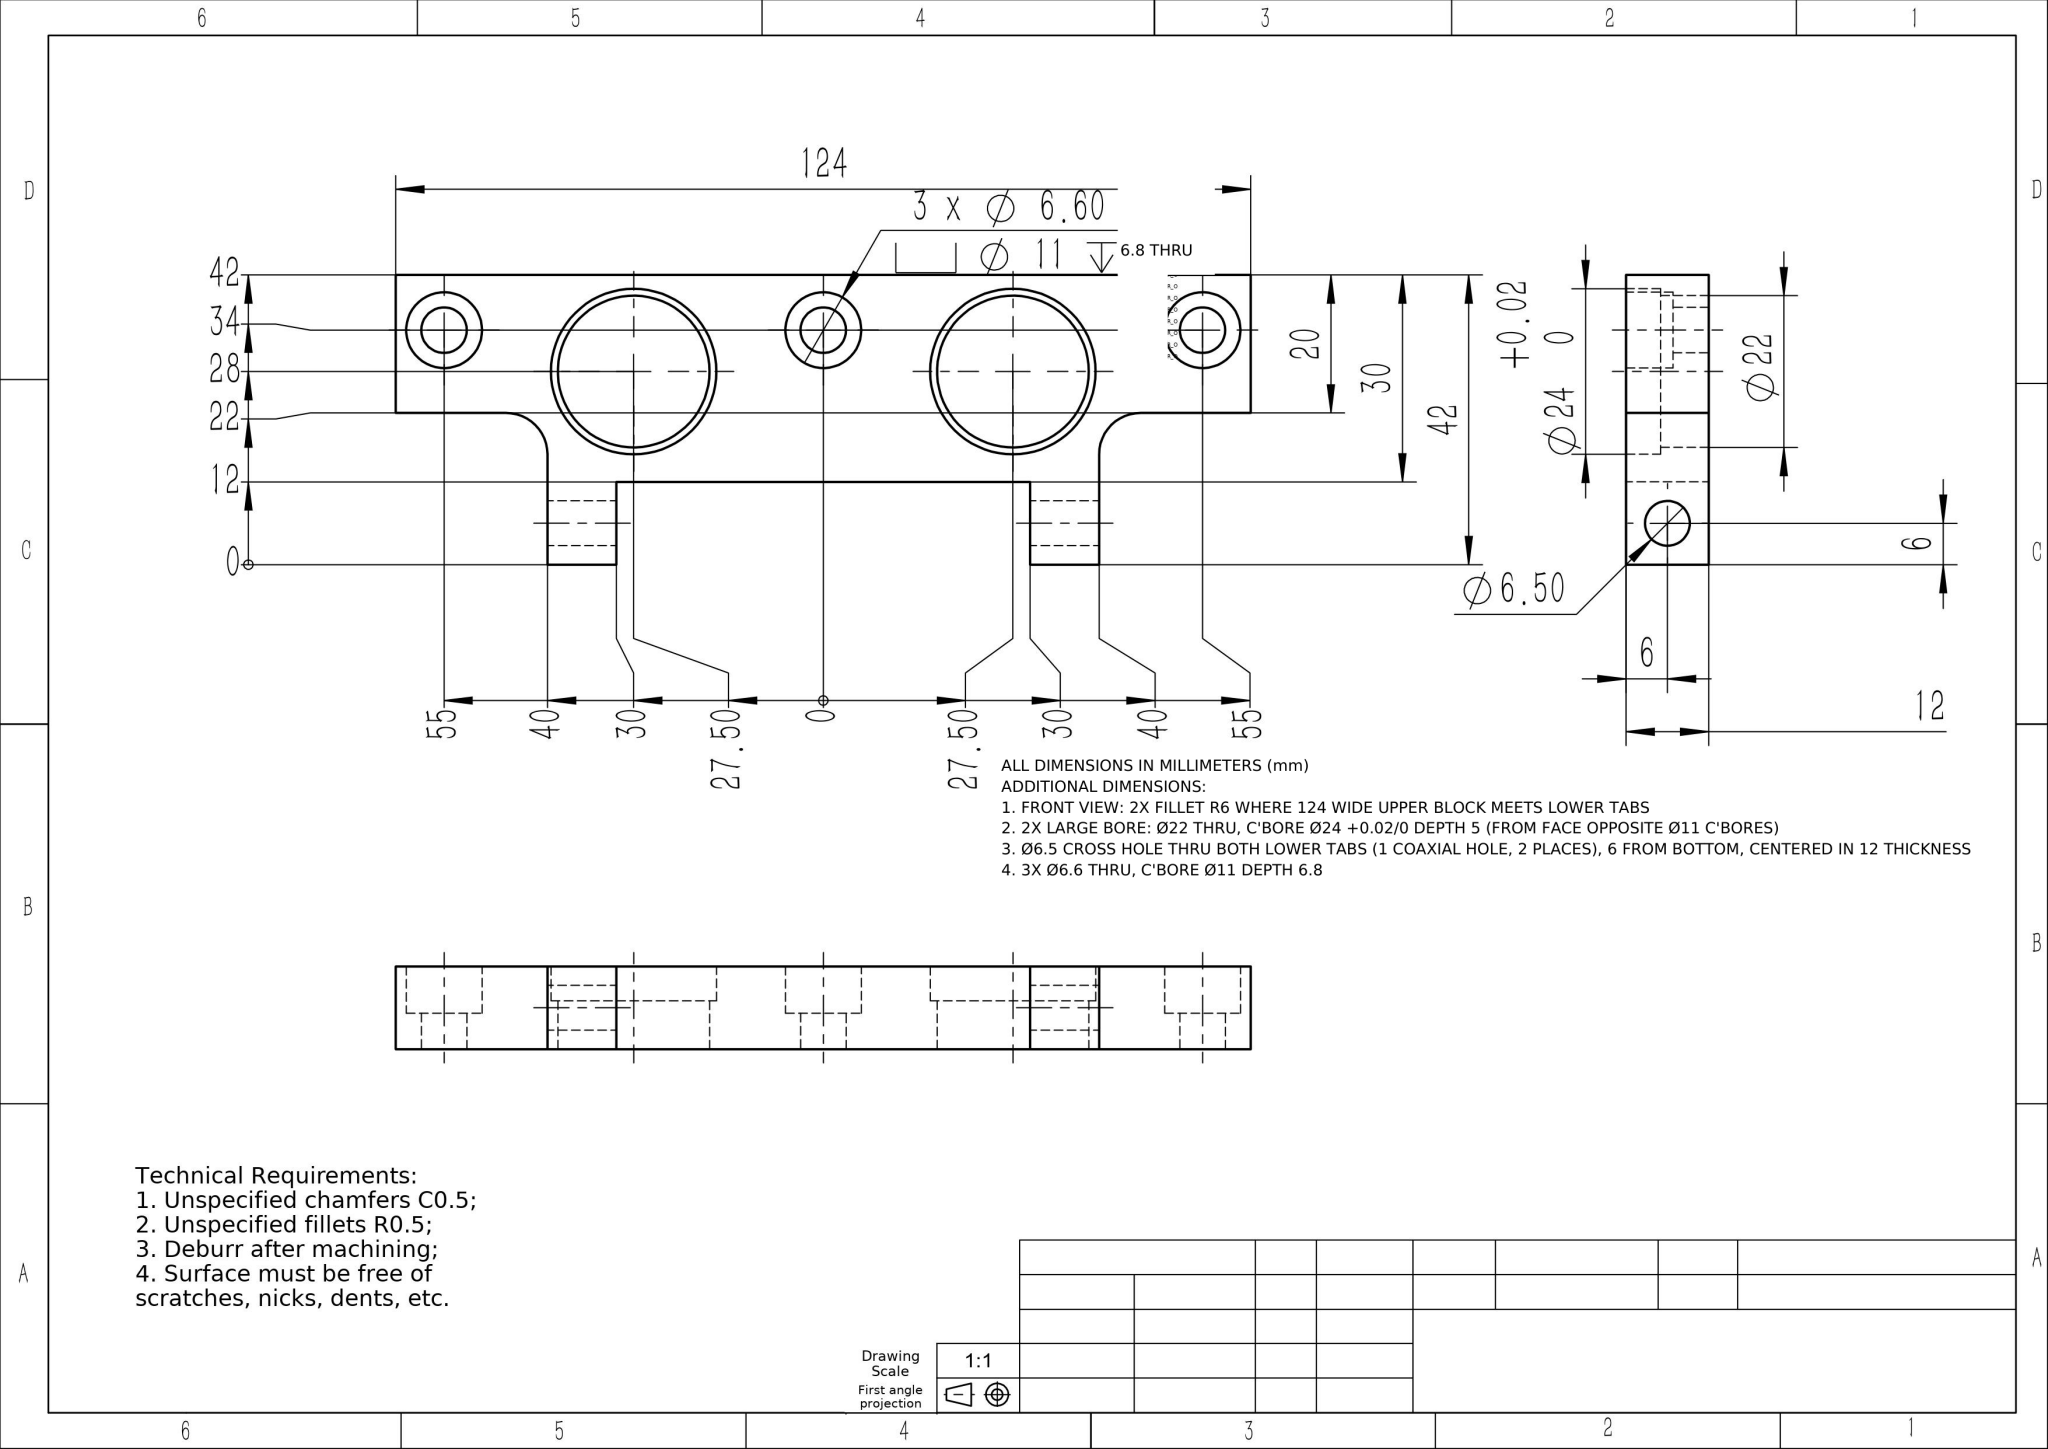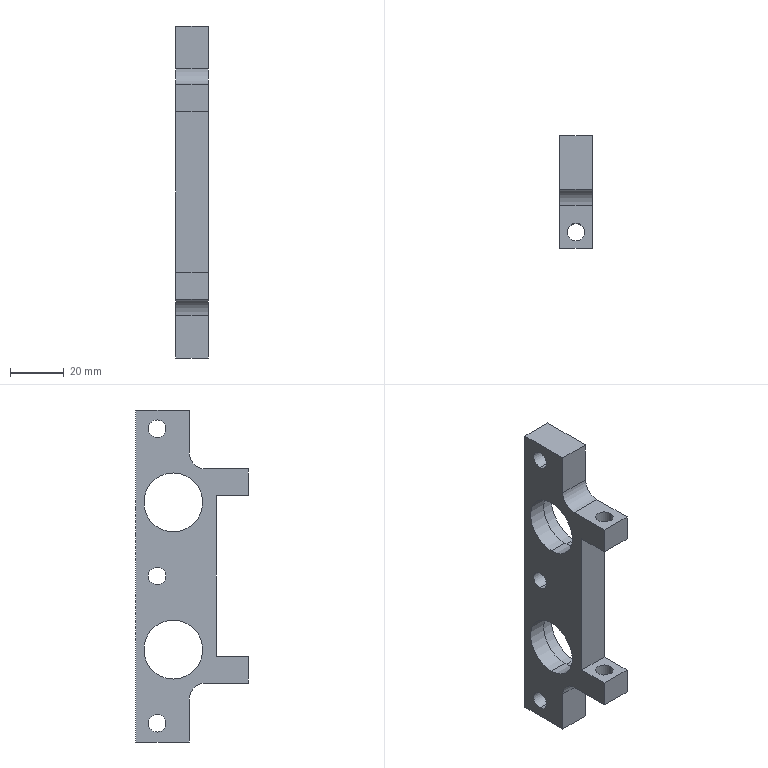Part | NX | mm | 1 solid | 45 faces | box 12 x 42 x 124 mm | volume 29444 mm3 | cylinder 26 | plane 19 | commonest cylinder face diameters 11 x6 6.6 x6 6.5 x4 22 x4 24 x4 12 x2